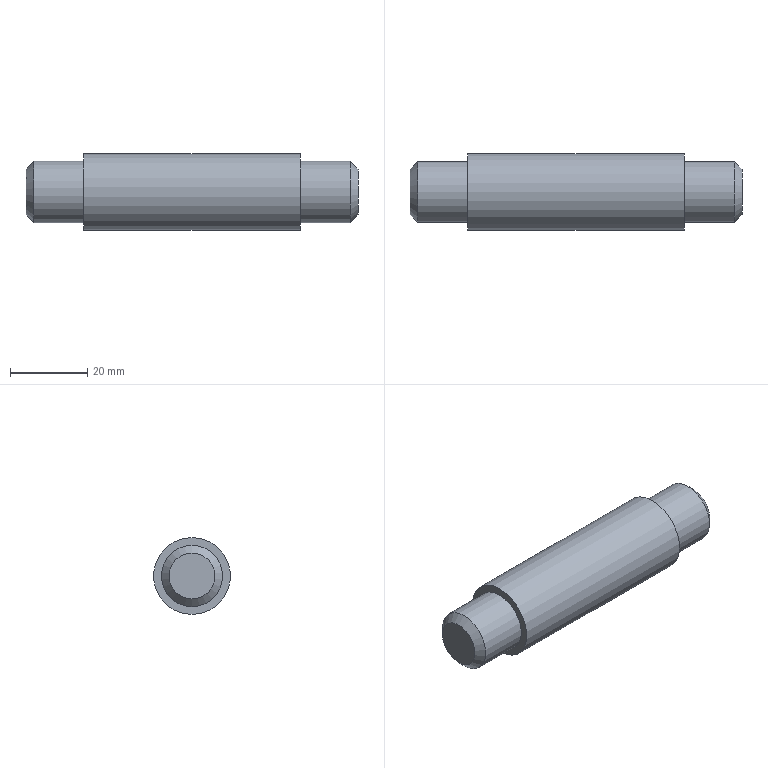Component | NX | EIXO_RODA | 1 solid | 9 faces | box 86 x 19.9 x 19.9 mm | volume 23191 mm3 | plane 4 | cylinder 3 | cone 2 | commonest cylinder face diameters 15.9 x2 19.9 x1
STEP:
#1=CARTESIAN_POINT('',(0.,0.,0.));
#2=DIRECTION('',(0.,0.,1.));
#3=DIRECTION('',(1.,0.,0.));
#4=AXIS2_PLACEMENT_3D('',#1,#2,#3);
#5=CARTESIAN_POINT('',(41.,0.,-17.95));
#6=VERTEX_POINT('',#5);
#7=CARTESIAN_POINT('',(41.,0.,-10.));
#8=DIRECTION('',(-1.,0.,0.));
#9=DIRECTION('',(0.,0.,-1.));
#10=AXIS2_PLACEMENT_3D('',#7,#8,#9);
#11=CIRCLE('',#10,7.95);
#12=CARTESIAN_POINT('',(43.,0.,-10.));
#13=DIRECTION('',(-1.,0.,0.));
#14=DIRECTION('',(0.,0.,-1.));
#15=AXIS2_PLACEMENT_3D('',#12,#13,#14);
#16=CYLINDRICAL_SURFACE('',#15,7.95);
#17=CARTESIAN_POINT('',(0.,2.));
#18=DIRECTION('',(1.,0.));
#19=VECTOR('',#18,1.);
#20=LINE('',#17,#19);
#21=(GEOMETRIC_REPRESENTATION_CONTEXT(2)PARAMETRIC_REPRESENTATION_CONTEXT()REPRESENTATION_CONTEXT('',''));
#22=DEFINITIONAL_REPRESENTATION('',(#20),#21);
#23=PCURVE('',#16,#22);
#24=CARTESIAN_POINT('',(43.,0.,-10.));
#25=DIRECTION('',(-1.,0.,0.));
#26=DIRECTION('',(0.,0.,-1.));
#27=AXIS2_PLACEMENT_3D('',#24,#25,#26);
#28=CONICAL_SURFACE('',#27,5.95,0.7854);
#29=CARTESIAN_POINT('',(0.,2.));
#30=DIRECTION('',(1.,0.));
#31=VECTOR('',#30,1.);
#32=LINE('',#29,#31);
#33=(GEOMETRIC_REPRESENTATION_CONTEXT(2)PARAMETRIC_REPRESENTATION_CONTEXT()REPRESENTATION_CONTEXT('',''));
#34=DEFINITIONAL_REPRESENTATION('',(#32),#33);
#35=PCURVE('',#28,#34);
#36=SURFACE_CURVE('',#11,(#23,#35),.PCURVE_S1.);
#37=EDGE_CURVE('',#6,#6,#36,.T.);
#38=ORIENTED_EDGE('',*,*,#37,.T.);
#39=CARTESIAN_POINT('',(28.,0.,-17.95));
#40=VERTEX_POINT('',#39);
#41=CARTESIAN_POINT('',(41.,0.,-17.95));
#42=CARTESIAN_POINT('',(28.,0.,-17.95));
#43=B_SPLINE_CURVE_WITH_KNOTS('',1,(#41,#42),.UNSPECIFIED.,.F.,.F.,(2,2),(2.,15.),.PIECEWISE_BEZIER_KNOTS.);
#44=CARTESIAN_POINT('',(6.283,0.));
#45=DIRECTION('',(0.,1.));
#46=VECTOR('',#45,1.);
#47=LINE('',#44,#46);
#48=(GEOMETRIC_REPRESENTATION_CONTEXT(2)PARAMETRIC_REPRESENTATION_CONTEXT()REPRESENTATION_CONTEXT('',''));
#49=DEFINITIONAL_REPRESENTATION('',(#47),#48);
#50=PCURVE('',#16,#49);
#51=CARTESIAN_POINT('',(0.,0.));
#52=DIRECTION('',(0.,1.));
#53=VECTOR('',#52,1.);
#54=LINE('',#51,#53);
#55=(GEOMETRIC_REPRESENTATION_CONTEXT(2)PARAMETRIC_REPRESENTATION_CONTEXT()REPRESENTATION_CONTEXT('',''));
#56=DEFINITIONAL_REPRESENTATION('',(#54),#55);
#57=PCURVE('',#16,#56);
#58=SEAM_CURVE('',#43,(#50,#57),.PCURVE_S1.);
#59=EDGE_CURVE('',#6,#40,#58,.T.);
#60=ORIENTED_EDGE('',*,*,#59,.T.);
#61=CARTESIAN_POINT('',(28.,0.,-2.05));
#62=VERTEX_POINT('',#61);
#63=CARTESIAN_POINT('',(28.,0.,-10.));
#64=DIRECTION('',(1.,0.,0.));
#65=DIRECTION('',(0.,0.,1.));
#66=AXIS2_PLACEMENT_3D('',#63,#64,#65);
#67=CIRCLE('',#66,7.95);
#68=CARTESIAN_POINT('',(9.425,15.));
#69=DIRECTION('',(-1.,0.));
#70=VECTOR('',#69,1.);
#71=LINE('',#68,#70);
#72=(GEOMETRIC_REPRESENTATION_CONTEXT(2)PARAMETRIC_REPRESENTATION_CONTEXT()REPRESENTATION_CONTEXT('',''));
#73=DEFINITIONAL_REPRESENTATION('',(#71),#72);
#74=PCURVE('',#16,#73);
#75=CARTESIAN_POINT('',(28.,0.,-10.));
#76=DIRECTION('',(1.,0.,0.));
#77=DIRECTION('',(0.,0.,1.));
#78=AXIS2_PLACEMENT_3D('',#75,#76,#77);
#79=PLANE('',#78);
#80=CARTESIAN_POINT('',(0.,0.));
#81=DIRECTION('',(1.,0.));
#82=AXIS2_PLACEMENT_2D('',#80,#81);
#83=CIRCLE('',#82,7.95);
#84=(GEOMETRIC_REPRESENTATION_CONTEXT(2)PARAMETRIC_REPRESENTATION_CONTEXT()REPRESENTATION_CONTEXT('',''));
#85=DEFINITIONAL_REPRESENTATION('',(#83),#84);
#86=PCURVE('',#79,#85);
#87=SURFACE_CURVE('',#67,(#74,#86),.PCURVE_S1.);
#88=EDGE_CURVE('',#40,#62,#87,.T.);
#89=ORIENTED_EDGE('',*,*,#88,.T.);
#90=CARTESIAN_POINT('',(28.,0.,-10.));
#91=DIRECTION('',(1.,0.,0.));
#92=DIRECTION('',(0.,0.,1.));
#93=AXIS2_PLACEMENT_3D('',#90,#91,#92);
#94=CIRCLE('',#93,7.95);
#95=CARTESIAN_POINT('',(3.142,15.));
#96=DIRECTION('',(-1.,0.));
#97=VECTOR('',#96,1.);
#98=LINE('',#95,#97);
#99=(GEOMETRIC_REPRESENTATION_CONTEXT(2)PARAMETRIC_REPRESENTATION_CONTEXT()REPRESENTATION_CONTEXT('',''));
#100=DEFINITIONAL_REPRESENTATION('',(#98),#99);
#101=PCURVE('',#16,#100);
#102=CARTESIAN_POINT('',(0.,0.));
#103=DIRECTION('',(1.,0.));
#104=AXIS2_PLACEMENT_2D('',#102,#103);
#105=CIRCLE('',#104,7.95);
#106=(GEOMETRIC_REPRESENTATION_CONTEXT(2)PARAMETRIC_REPRESENTATION_CONTEXT()REPRESENTATION_CONTEXT('',''));
#107=DEFINITIONAL_REPRESENTATION('',(#105),#106);
#108=PCURVE('',#79,#107);
#109=SURFACE_CURVE('',#94,(#101,#108),.PCURVE_S1.);
#110=EDGE_CURVE('',#62,#40,#109,.T.);
#111=ORIENTED_EDGE('',*,*,#110,.T.);
#112=ORIENTED_EDGE('',*,*,#59,.F.);
#113=EDGE_LOOP('',(#38,#60,#89,#111,#112));
#114=FACE_BOUND('',#113,.T.);
#115=ADVANCED_FACE('',(#114),#16,.T.);
#116=CARTESIAN_POINT('',(28.,0.,-0.05));
#117=VERTEX_POINT('',#116);
#118=CARTESIAN_POINT('',(28.,0.,-10.));
#119=DIRECTION('',(1.,0.,0.));
#120=DIRECTION('',(0.,0.,1.));
#121=AXIS2_PLACEMENT_3D('',#118,#119,#120);
#122=CIRCLE('',#121,9.95);
#123=CARTESIAN_POINT('',(28.,0.,-10.));
#124=DIRECTION('',(-1.,0.,0.));
#125=DIRECTION('',(0.,0.,-1.));
#126=AXIS2_PLACEMENT_3D('',#123,#124,#125);
#127=CYLINDRICAL_SURFACE('',#126,9.95);
#128=CARTESIAN_POINT('',(9.425,0.));
#129=DIRECTION('',(-1.,0.));
#130=VECTOR('',#129,1.);
#131=LINE('',#128,#130);
#132=(GEOMETRIC_REPRESENTATION_CONTEXT(2)PARAMETRIC_REPRESENTATION_CONTEXT()REPRESENTATION_CONTEXT('',''));
#133=DEFINITIONAL_REPRESENTATION('',(#131),#132);
#134=PCURVE('',#127,#133);
#135=CARTESIAN_POINT('',(0.,0.));
#136=DIRECTION('',(1.,0.));
#137=AXIS2_PLACEMENT_2D('',#135,#136);
#138=CIRCLE('',#137,9.95);
#139=(GEOMETRIC_REPRESENTATION_CONTEXT(2)PARAMETRIC_REPRESENTATION_CONTEXT()REPRESENTATION_CONTEXT('',''));
#140=DEFINITIONAL_REPRESENTATION('',(#138),#139);
#141=PCURVE('',#79,#140);
#142=SURFACE_CURVE('',#122,(#134,#141),.PCURVE_S1.);
#143=EDGE_CURVE('',#117,#117,#142,.T.);
#144=ORIENTED_EDGE('',*,*,#143,.F.);
#145=CARTESIAN_POINT('',(-28.,0.,-0.05));
#146=VERTEX_POINT('',#145);
#147=CARTESIAN_POINT('',(28.,0.,-0.05));
#148=CARTESIAN_POINT('',(-28.,0.,-0.05));
#149=B_SPLINE_CURVE_WITH_KNOTS('',1,(#147,#148),.UNSPECIFIED.,.F.,.F.,(2,2),(0.,56.),.PIECEWISE_BEZIER_KNOTS.);
#150=CARTESIAN_POINT('',(9.425,0.));
#151=DIRECTION('',(0.,1.));
#152=VECTOR('',#151,1.);
#153=LINE('',#150,#152);
#154=(GEOMETRIC_REPRESENTATION_CONTEXT(2)PARAMETRIC_REPRESENTATION_CONTEXT()REPRESENTATION_CONTEXT('',''));
#155=DEFINITIONAL_REPRESENTATION('',(#153),#154);
#156=PCURVE('',#127,#155);
#157=CARTESIAN_POINT('',(3.142,0.));
#158=DIRECTION('',(0.,1.));
#159=VECTOR('',#158,1.);
#160=LINE('',#157,#159);
#161=(GEOMETRIC_REPRESENTATION_CONTEXT(2)PARAMETRIC_REPRESENTATION_CONTEXT()REPRESENTATION_CONTEXT('',''));
#162=DEFINITIONAL_REPRESENTATION('',(#160),#161);
#163=PCURVE('',#127,#162);
#164=SEAM_CURVE('',#149,(#156,#163),.PCURVE_S1.);
#165=EDGE_CURVE('',#117,#146,#164,.T.);
#166=ORIENTED_EDGE('',*,*,#165,.T.);
#167=CARTESIAN_POINT('',(-28.,0.,-10.));
#168=DIRECTION('',(1.,0.,0.));
#169=DIRECTION('',(0.,0.,1.));
#170=AXIS2_PLACEMENT_3D('',#167,#168,#169);
#171=CIRCLE('',#170,9.95);
#172=CARTESIAN_POINT('',(9.425,56.));
#173=DIRECTION('',(-1.,0.));
#174=VECTOR('',#173,1.);
#175=LINE('',#172,#174);
#176=(GEOMETRIC_REPRESENTATION_CONTEXT(2)PARAMETRIC_REPRESENTATION_CONTEXT()REPRESENTATION_CONTEXT('',''));
#177=DEFINITIONAL_REPRESENTATION('',(#175),#176);
#178=PCURVE('',#127,#177);
#179=CARTESIAN_POINT('',(-28.,0.,-10.));
#180=DIRECTION('',(1.,0.,0.));
#181=DIRECTION('',(0.,0.,1.));
#182=AXIS2_PLACEMENT_3D('',#179,#180,#181);
#183=PLANE('',#182);
#184=CARTESIAN_POINT('',(0.,0.));
#185=DIRECTION('',(1.,0.));
#186=AXIS2_PLACEMENT_2D('',#184,#185);
#187=CIRCLE('',#186,9.95);
#188=(GEOMETRIC_REPRESENTATION_CONTEXT(2)PARAMETRIC_REPRESENTATION_CONTEXT()REPRESENTATION_CONTEXT('',''));
#189=DEFINITIONAL_REPRESENTATION('',(#187),#188);
#190=PCURVE('',#183,#189);
#191=SURFACE_CURVE('',#171,(#178,#190),.PCURVE_S1.);
#192=EDGE_CURVE('',#146,#146,#191,.T.);
#193=ORIENTED_EDGE('',*,*,#192,.T.);
#194=ORIENTED_EDGE('',*,*,#165,.F.);
#195=EDGE_LOOP('',(#144,#166,#193,#194));
#196=FACE_BOUND('',#195,.T.);
#197=ADVANCED_FACE('',(#196),#127,.T.);
#198=ORIENTED_EDGE('',*,*,#143,.T.);
#199=EDGE_LOOP('',(#198));
#200=FACE_BOUND('',#199,.T.);
#201=ORIENTED_EDGE('',*,*,#110,.F.);
#202=ORIENTED_EDGE('',*,*,#88,.F.);
#203=EDGE_LOOP('',(#201,#202));
#204=FACE_BOUND('',#203,.T.);
#205=ADVANCED_FACE('',(#200,#204),#79,.T.);
#206=ORIENTED_EDGE('',*,*,#192,.F.);
#207=EDGE_LOOP('',(#206));
#208=FACE_BOUND('',#207,.T.);
#209=CARTESIAN_POINT('',(-28.,0.,-2.05));
#210=VERTEX_POINT('',#209);
#211=CARTESIAN_POINT('',(-28.,0.,-17.95));
#212=VERTEX_POINT('',#211);
#213=CARTESIAN_POINT('',(-28.,0.,-10.));
#214=DIRECTION('',(1.,0.,0.));
#215=DIRECTION('',(0.,0.,1.));
#216=AXIS2_PLACEMENT_3D('',#213,#214,#215);
#217=CIRCLE('',#216,7.95);
#218=CARTESIAN_POINT('',(0.,0.));
#219=DIRECTION('',(1.,0.));
#220=AXIS2_PLACEMENT_2D('',#218,#219);
#221=CIRCLE('',#220,7.95);
#222=(GEOMETRIC_REPRESENTATION_CONTEXT(2)PARAMETRIC_REPRESENTATION_CONTEXT()REPRESENTATION_CONTEXT('',''));
#223=DEFINITIONAL_REPRESENTATION('',(#221),#222);
#224=PCURVE('',#183,#223);
#225=CARTESIAN_POINT('',(43.,0.,-10.));
#226=DIRECTION('',(-1.,0.,0.));
#227=DIRECTION('',(0.,0.,-1.));
#228=AXIS2_PLACEMENT_3D('',#225,#226,#227);
#229=CYLINDRICAL_SURFACE('',#228,7.95);
#230=CARTESIAN_POINT('',(3.142,71.));
#231=DIRECTION('',(-1.,0.));
#232=VECTOR('',#231,1.);
#233=LINE('',#230,#232);
#234=(GEOMETRIC_REPRESENTATION_CONTEXT(2)PARAMETRIC_REPRESENTATION_CONTEXT()REPRESENTATION_CONTEXT('',''));
#235=DEFINITIONAL_REPRESENTATION('',(#233),#234);
#236=PCURVE('',#229,#235);
#237=SURFACE_CURVE('',#217,(#224,#236),.PCURVE_S1.);
#238=EDGE_CURVE('',#210,#212,#237,.T.);
#239=ORIENTED_EDGE('',*,*,#238,.T.);
#240=CARTESIAN_POINT('',(-28.,0.,-10.));
#241=DIRECTION('',(1.,0.,0.));
#242=DIRECTION('',(0.,0.,1.));
#243=AXIS2_PLACEMENT_3D('',#240,#241,#242);
#244=CIRCLE('',#243,7.95);
#245=CARTESIAN_POINT('',(0.,0.));
#246=DIRECTION('',(1.,0.));
#247=AXIS2_PLACEMENT_2D('',#245,#246);
#248=CIRCLE('',#247,7.95);
#249=(GEOMETRIC_REPRESENTATION_CONTEXT(2)PARAMETRIC_REPRESENTATION_CONTEXT()REPRESENTATION_CONTEXT('',''));
#250=DEFINITIONAL_REPRESENTATION('',(#248),#249);
#251=PCURVE('',#183,#250);
#252=CARTESIAN_POINT('',(9.425,71.));
#253=DIRECTION('',(-1.,0.));
#254=VECTOR('',#253,1.);
#255=LINE('',#252,#254);
#256=(GEOMETRIC_REPRESENTATION_CONTEXT(2)PARAMETRIC_REPRESENTATION_CONTEXT()REPRESENTATION_CONTEXT('',''));
#257=DEFINITIONAL_REPRESENTATION('',(#255),#256);
#258=PCURVE('',#229,#257);
#259=SURFACE_CURVE('',#244,(#251,#258),.PCURVE_S1.);
#260=EDGE_CURVE('',#212,#210,#259,.T.);
#261=ORIENTED_EDGE('',*,*,#260,.T.);
#262=EDGE_LOOP('',(#239,#261));
#263=FACE_BOUND('',#262,.T.);
#264=ADVANCED_FACE('',(#208,#263),#183,.F.);
#265=CARTESIAN_POINT('',(-41.,0.,-17.95));
#266=VERTEX_POINT('',#265);
#267=CARTESIAN_POINT('',(-41.,0.,-10.));
#268=DIRECTION('',(-1.,0.,0.));
#269=DIRECTION('',(0.,0.,-1.));
#270=AXIS2_PLACEMENT_3D('',#267,#268,#269);
#271=CIRCLE('',#270,7.95);
#272=CARTESIAN_POINT('',(0.,84.));
#273=DIRECTION('',(1.,0.));
#274=VECTOR('',#273,1.);
#275=LINE('',#272,#274);
#276=(GEOMETRIC_REPRESENTATION_CONTEXT(2)PARAMETRIC_REPRESENTATION_CONTEXT()REPRESENTATION_CONTEXT('',''));
#277=DEFINITIONAL_REPRESENTATION('',(#275),#276);
#278=PCURVE('',#229,#277);
#279=CARTESIAN_POINT('',(-41.,0.,-10.));
#280=DIRECTION('',(1.,0.,0.));
#281=DIRECTION('',(0.,0.,1.));
#282=AXIS2_PLACEMENT_3D('',#279,#280,#281);
#283=CONICAL_SURFACE('',#282,7.95,0.7854);
#284=CARTESIAN_POINT('',(9.425,0.));
#285=DIRECTION('',(-1.,0.));
#286=VECTOR('',#285,1.);
#287=LINE('',#284,#286);
#288=(GEOMETRIC_REPRESENTATION_CONTEXT(2)PARAMETRIC_REPRESENTATION_CONTEXT()REPRESENTATION_CONTEXT('',''));
#289=DEFINITIONAL_REPRESENTATION('',(#287),#288);
#290=PCURVE('',#283,#289);
#291=SURFACE_CURVE('',#271,(#278,#290),.PCURVE_S1.);
#292=EDGE_CURVE('',#266,#266,#291,.T.);
#293=ORIENTED_EDGE('',*,*,#292,.F.);
#294=CARTESIAN_POINT('',(-28.,0.,-17.95));
#295=CARTESIAN_POINT('',(-41.,0.,-17.95));
#296=B_SPLINE_CURVE_WITH_KNOTS('',1,(#294,#295),.UNSPECIFIED.,.F.,.F.,(2,2),(71.,84.),.PIECEWISE_BEZIER_KNOTS.);
#297=CARTESIAN_POINT('',(0.,0.));
#298=DIRECTION('',(0.,1.));
#299=VECTOR('',#298,1.);
#300=LINE('',#297,#299);
#301=(GEOMETRIC_REPRESENTATION_CONTEXT(2)PARAMETRIC_REPRESENTATION_CONTEXT()REPRESENTATION_CONTEXT('',''));
#302=DEFINITIONAL_REPRESENTATION('',(#300),#301);
#303=PCURVE('',#229,#302);
#304=CARTESIAN_POINT('',(6.283,0.));
#305=DIRECTION('',(0.,1.));
#306=VECTOR('',#305,1.);
#307=LINE('',#304,#306);
#308=(GEOMETRIC_REPRESENTATION_CONTEXT(2)PARAMETRIC_REPRESENTATION_CONTEXT()REPRESENTATION_CONTEXT('',''));
#309=DEFINITIONAL_REPRESENTATION('',(#307),#308);
#310=PCURVE('',#229,#309);
#311=SEAM_CURVE('',#296,(#303,#310),.PCURVE_S1.);
#312=EDGE_CURVE('',#212,#266,#311,.T.);
#313=ORIENTED_EDGE('',*,*,#312,.F.);
#314=ORIENTED_EDGE('',*,*,#238,.F.);
#315=ORIENTED_EDGE('',*,*,#260,.F.);
#316=ORIENTED_EDGE('',*,*,#312,.T.);
#317=EDGE_LOOP('',(#293,#313,#314,#315,#316));
#318=FACE_BOUND('',#317,.T.);
#319=ADVANCED_FACE('',(#318),#229,.T.);
#320=CARTESIAN_POINT('',(-43.,0.,-15.95));
#321=VERTEX_POINT('',#320);
#322=CARTESIAN_POINT('',(-43.,0.,-10.));
#323=DIRECTION('',(-1.,0.,0.));
#324=DIRECTION('',(0.,0.,-1.));
#325=AXIS2_PLACEMENT_3D('',#322,#323,#324);
#326=CIRCLE('',#325,5.95);
#327=CARTESIAN_POINT('',(9.425,-2.));
#328=DIRECTION('',(-1.,0.));
#329=VECTOR('',#328,1.);
#330=LINE('',#327,#329);
#331=(GEOMETRIC_REPRESENTATION_CONTEXT(2)PARAMETRIC_REPRESENTATION_CONTEXT()REPRESENTATION_CONTEXT('',''));
#332=DEFINITIONAL_REPRESENTATION('',(#330),#331);
#333=PCURVE('',#283,#332);
#334=CARTESIAN_POINT('',(-43.,0.,-10.));
#335=DIRECTION('',(1.,0.,0.));
#336=DIRECTION('',(0.,0.,1.));
#337=AXIS2_PLACEMENT_3D('',#334,#335,#336);
#338=PLANE('',#337);
#339=CARTESIAN_POINT('',(-5.95,0.));
#340=CARTESIAN_POINT('',(-5.95,10.306));
#341=CARTESIAN_POINT('',(2.975,5.153));
#342=CARTESIAN_POINT('',(11.9,0.));
#343=CARTESIAN_POINT('',(2.975,-5.153));
#344=CARTESIAN_POINT('',(-5.95,-10.306));
#345=CARTESIAN_POINT('',(-5.95,0.));
#346=(BOUNDED_CURVE()B_SPLINE_CURVE(2,(#339,#340,#341,#342,#343,#344,#345),.UNSPECIFIED.,.T.,.F.)B_SPLINE_CURVE_WITH_KNOTS((1,2,2,2,2,1),(-2.094,0.,2.094,4.189,6.283,8.378),.UNSPECIFIED.)CURVE()GEOMETRIC_REPRESENTATION_ITEM()RATIONAL_B_SPLINE_CURVE((1.,0.5,1.,0.5,1.,0.5,1.))REPRESENTATION_ITEM(''));
#347=(GEOMETRIC_REPRESENTATION_CONTEXT(2)PARAMETRIC_REPRESENTATION_CONTEXT()REPRESENTATION_CONTEXT('',''));
#348=DEFINITIONAL_REPRESENTATION('',(#346),#347);
#349=PCURVE('',#338,#348);
#350=SURFACE_CURVE('',#326,(#333,#349),.PCURVE_S1.);
#351=EDGE_CURVE('',#321,#321,#350,.T.);
#352=ORIENTED_EDGE('',*,*,#351,.F.);
#353=CARTESIAN_POINT('',(-43.,0.,-15.95));
#354=CARTESIAN_POINT('',(-41.,0.,-17.95));
#355=B_SPLINE_CURVE_WITH_KNOTS('',1,(#353,#354),.UNSPECIFIED.,.F.,.F.,(2,2),(-2.828,0.),.PIECEWISE_BEZIER_KNOTS.);
#356=CARTESIAN_POINT('',(9.425,0.));
#357=DIRECTION('',(0.,1.));
#358=VECTOR('',#357,1.);
#359=LINE('',#356,#358);
#360=(GEOMETRIC_REPRESENTATION_CONTEXT(2)PARAMETRIC_REPRESENTATION_CONTEXT()REPRESENTATION_CONTEXT('',''));
#361=DEFINITIONAL_REPRESENTATION('',(#359),#360);
#362=PCURVE('',#283,#361);
#363=CARTESIAN_POINT('',(3.142,0.));
#364=DIRECTION('',(0.,1.));
#365=VECTOR('',#364,1.);
#366=LINE('',#363,#365);
#367=(GEOMETRIC_REPRESENTATION_CONTEXT(2)PARAMETRIC_REPRESENTATION_CONTEXT()REPRESENTATION_CONTEXT('',''));
#368=DEFINITIONAL_REPRESENTATION('',(#366),#367);
#369=PCURVE('',#283,#368);
#370=SEAM_CURVE('',#355,(#362,#369),.PCURVE_S1.);
#371=EDGE_CURVE('',#321,#266,#370,.T.);
#372=ORIENTED_EDGE('',*,*,#371,.T.);
#373=ORIENTED_EDGE('',*,*,#292,.T.);
#374=ORIENTED_EDGE('',*,*,#371,.F.);
#375=EDGE_LOOP('',(#352,#372,#373,#374));
#376=FACE_BOUND('',#375,.T.);
#377=ADVANCED_FACE('',(#376),#283,.T.);
#378=ORIENTED_EDGE('',*,*,#351,.T.);
#379=EDGE_LOOP('',(#378));
#380=FACE_BOUND('',#379,.T.);
#381=ADVANCED_FACE('',(#380),#338,.F.);
#382=ORIENTED_EDGE('',*,*,#37,.F.);
#383=CARTESIAN_POINT('',(43.,0.,-15.95));
#384=VERTEX_POINT('',#383);
#385=CARTESIAN_POINT('',(43.,0.,-15.95));
#386=CARTESIAN_POINT('',(41.,0.,-17.95));
#387=B_SPLINE_CURVE_WITH_KNOTS('',1,(#385,#386),.UNSPECIFIED.,.F.,.F.,(2,2),(0.,2.828),.PIECEWISE_BEZIER_KNOTS.);
#388=CARTESIAN_POINT('',(0.,0.));
#389=DIRECTION('',(0.,1.));
#390=VECTOR('',#389,1.);
#391=LINE('',#388,#390);
#392=(GEOMETRIC_REPRESENTATION_CONTEXT(2)PARAMETRIC_REPRESENTATION_CONTEXT()REPRESENTATION_CONTEXT('',''));
#393=DEFINITIONAL_REPRESENTATION('',(#391),#392);
#394=PCURVE('',#28,#393);
#395=CARTESIAN_POINT('',(6.283,0.));
#396=DIRECTION('',(0.,1.));
#397=VECTOR('',#396,1.);
#398=LINE('',#395,#397);
#399=(GEOMETRIC_REPRESENTATION_CONTEXT(2)PARAMETRIC_REPRESENTATION_CONTEXT()REPRESENTATION_CONTEXT('',''));
#400=DEFINITIONAL_REPRESENTATION('',(#398),#399);
#401=PCURVE('',#28,#400);
#402=SEAM_CURVE('',#387,(#394,#401),.PCURVE_S1.);
#403=EDGE_CURVE('',#384,#6,#402,.T.);
#404=ORIENTED_EDGE('',*,*,#403,.F.);
#405=CARTESIAN_POINT('',(43.,0.,-10.));
#406=DIRECTION('',(-1.,0.,0.));
#407=DIRECTION('',(0.,0.,-1.));
#408=AXIS2_PLACEMENT_3D('',#405,#406,#407);
#409=CIRCLE('',#408,5.95);
#410=CARTESIAN_POINT('',(0.,0.));
#411=DIRECTION('',(1.,0.));
#412=VECTOR('',#411,1.);
#413=LINE('',#410,#412);
#414=(GEOMETRIC_REPRESENTATION_CONTEXT(2)PARAMETRIC_REPRESENTATION_CONTEXT()REPRESENTATION_CONTEXT('',''));
#415=DEFINITIONAL_REPRESENTATION('',(#413),#414);
#416=PCURVE('',#28,#415);
#417=CARTESIAN_POINT('',(43.,0.,-10.));
#418=DIRECTION('',(1.,0.,0.));
#419=DIRECTION('',(0.,0.,1.));
#420=AXIS2_PLACEMENT_3D('',#417,#418,#419);
#421=PLANE('',#420);
#422=CARTESIAN_POINT('',(-5.95,0.));
#423=CARTESIAN_POINT('',(-5.95,10.306));
#424=CARTESIAN_POINT('',(2.975,5.153));
#425=CARTESIAN_POINT('',(11.9,0.));
#426=CARTESIAN_POINT('',(2.975,-5.153));
#427=CARTESIAN_POINT('',(-5.95,-10.306));
#428=CARTESIAN_POINT('',(-5.95,0.));
#429=(BOUNDED_CURVE()B_SPLINE_CURVE(2,(#422,#423,#424,#425,#426,#427,#428),.UNSPECIFIED.,.T.,.F.)B_SPLINE_CURVE_WITH_KNOTS((1,2,2,2,2,1),(-2.094,0.,2.094,4.189,6.283,8.378),.UNSPECIFIED.)CURVE()GEOMETRIC_REPRESENTATION_ITEM()RATIONAL_B_SPLINE_CURVE((1.,0.5,1.,0.5,1.,0.5,1.))REPRESENTATION_ITEM(''));
#430=(GEOMETRIC_REPRESENTATION_CONTEXT(2)PARAMETRIC_REPRESENTATION_CONTEXT()REPRESENTATION_CONTEXT('',''));
#431=DEFINITIONAL_REPRESENTATION('',(#429),#430);
#432=PCURVE('',#421,#431);
#433=SURFACE_CURVE('',#409,(#416,#432),.PCURVE_S1.);
#434=EDGE_CURVE('',#384,#384,#433,.T.);
#435=ORIENTED_EDGE('',*,*,#434,.T.);
#436=ORIENTED_EDGE('',*,*,#403,.T.);
#437=EDGE_LOOP('',(#382,#404,#435,#436));
#438=FACE_BOUND('',#437,.T.);
#439=ADVANCED_FACE('',(#438),#28,.T.);
#440=ORIENTED_EDGE('',*,*,#434,.F.);
#441=EDGE_LOOP('',(#440));
#442=FACE_BOUND('',#441,.T.);
#443=ADVANCED_FACE('',(#442),#421,.T.);
#444=CLOSED_SHELL('',(#115,#197,#205,#264,#319,#377,#381,#439,#443));
#445=MANIFOLD_SOLID_BREP('',#444);
#446=(LENGTH_UNIT()NAMED_UNIT(*)SI_UNIT(.MILLI.,.METRE.));
#447=UNCERTAINTY_MEASURE_WITH_UNIT(LENGTH_MEASURE(0.000005),#446,'','');
#448=(NAMED_UNIT(*)PLANE_ANGLE_UNIT()SI_UNIT($,.RADIAN.));
#449=(NAMED_UNIT(*)SI_UNIT($,.STERADIAN.)SOLID_ANGLE_UNIT());
#450=(GEOMETRIC_REPRESENTATION_CONTEXT(3)GLOBAL_UNCERTAINTY_ASSIGNED_CONTEXT((#447))GLOBAL_UNIT_ASSIGNED_CONTEXT((#446,#448,#449))REPRESENTATION_CONTEXT('',''));
#451=ADVANCED_BREP_SHAPE_REPRESENTATION('',(#4,#445),#450);